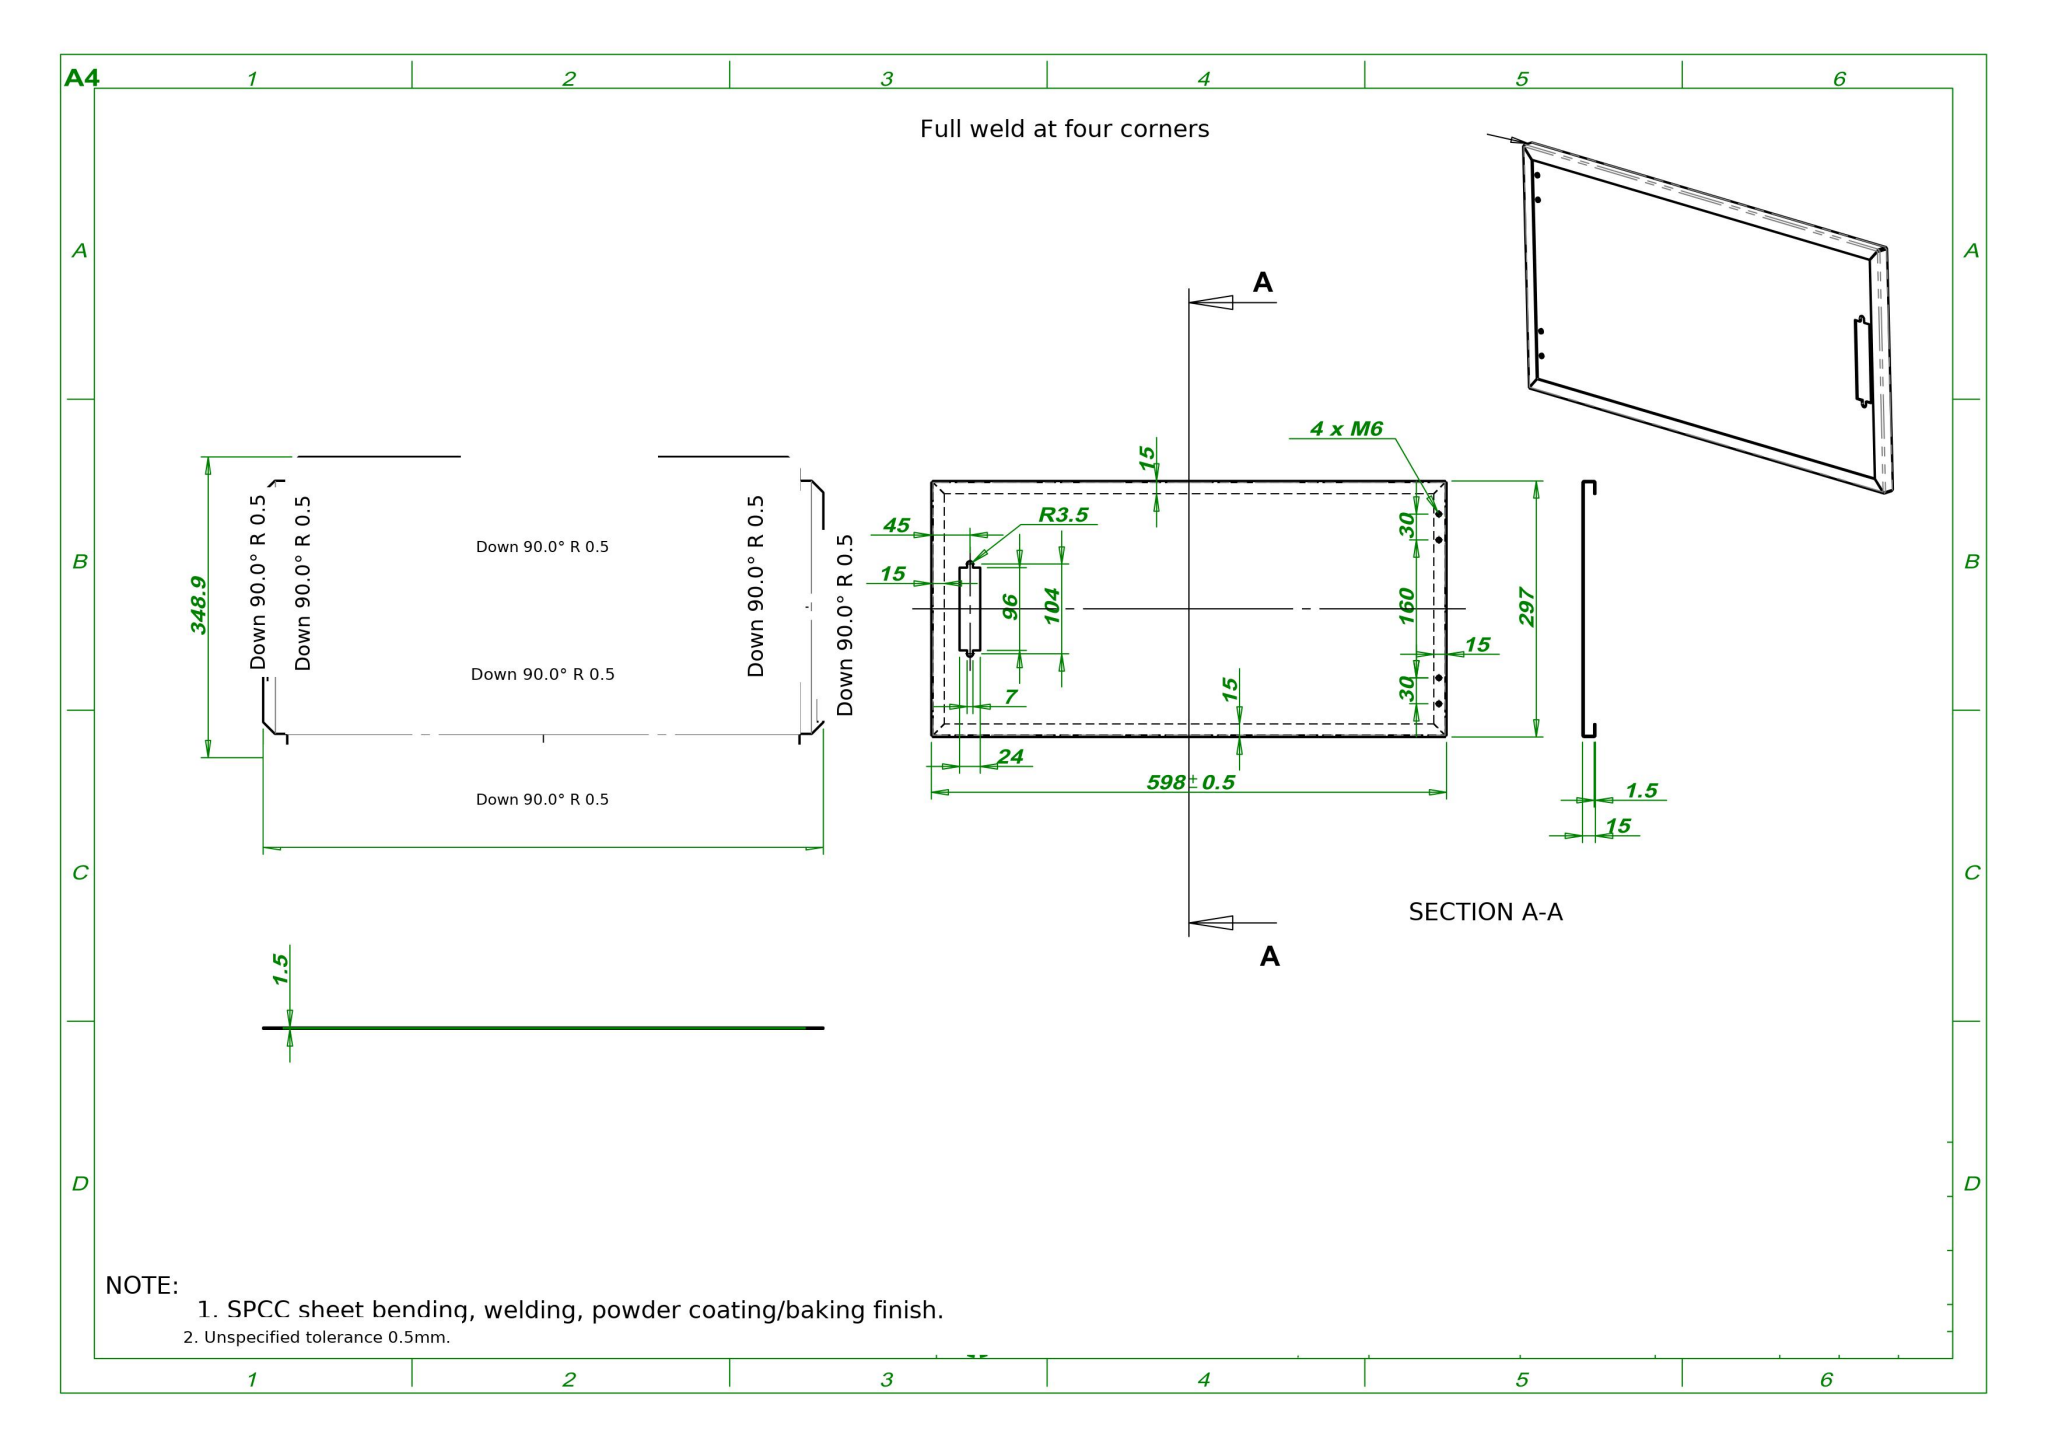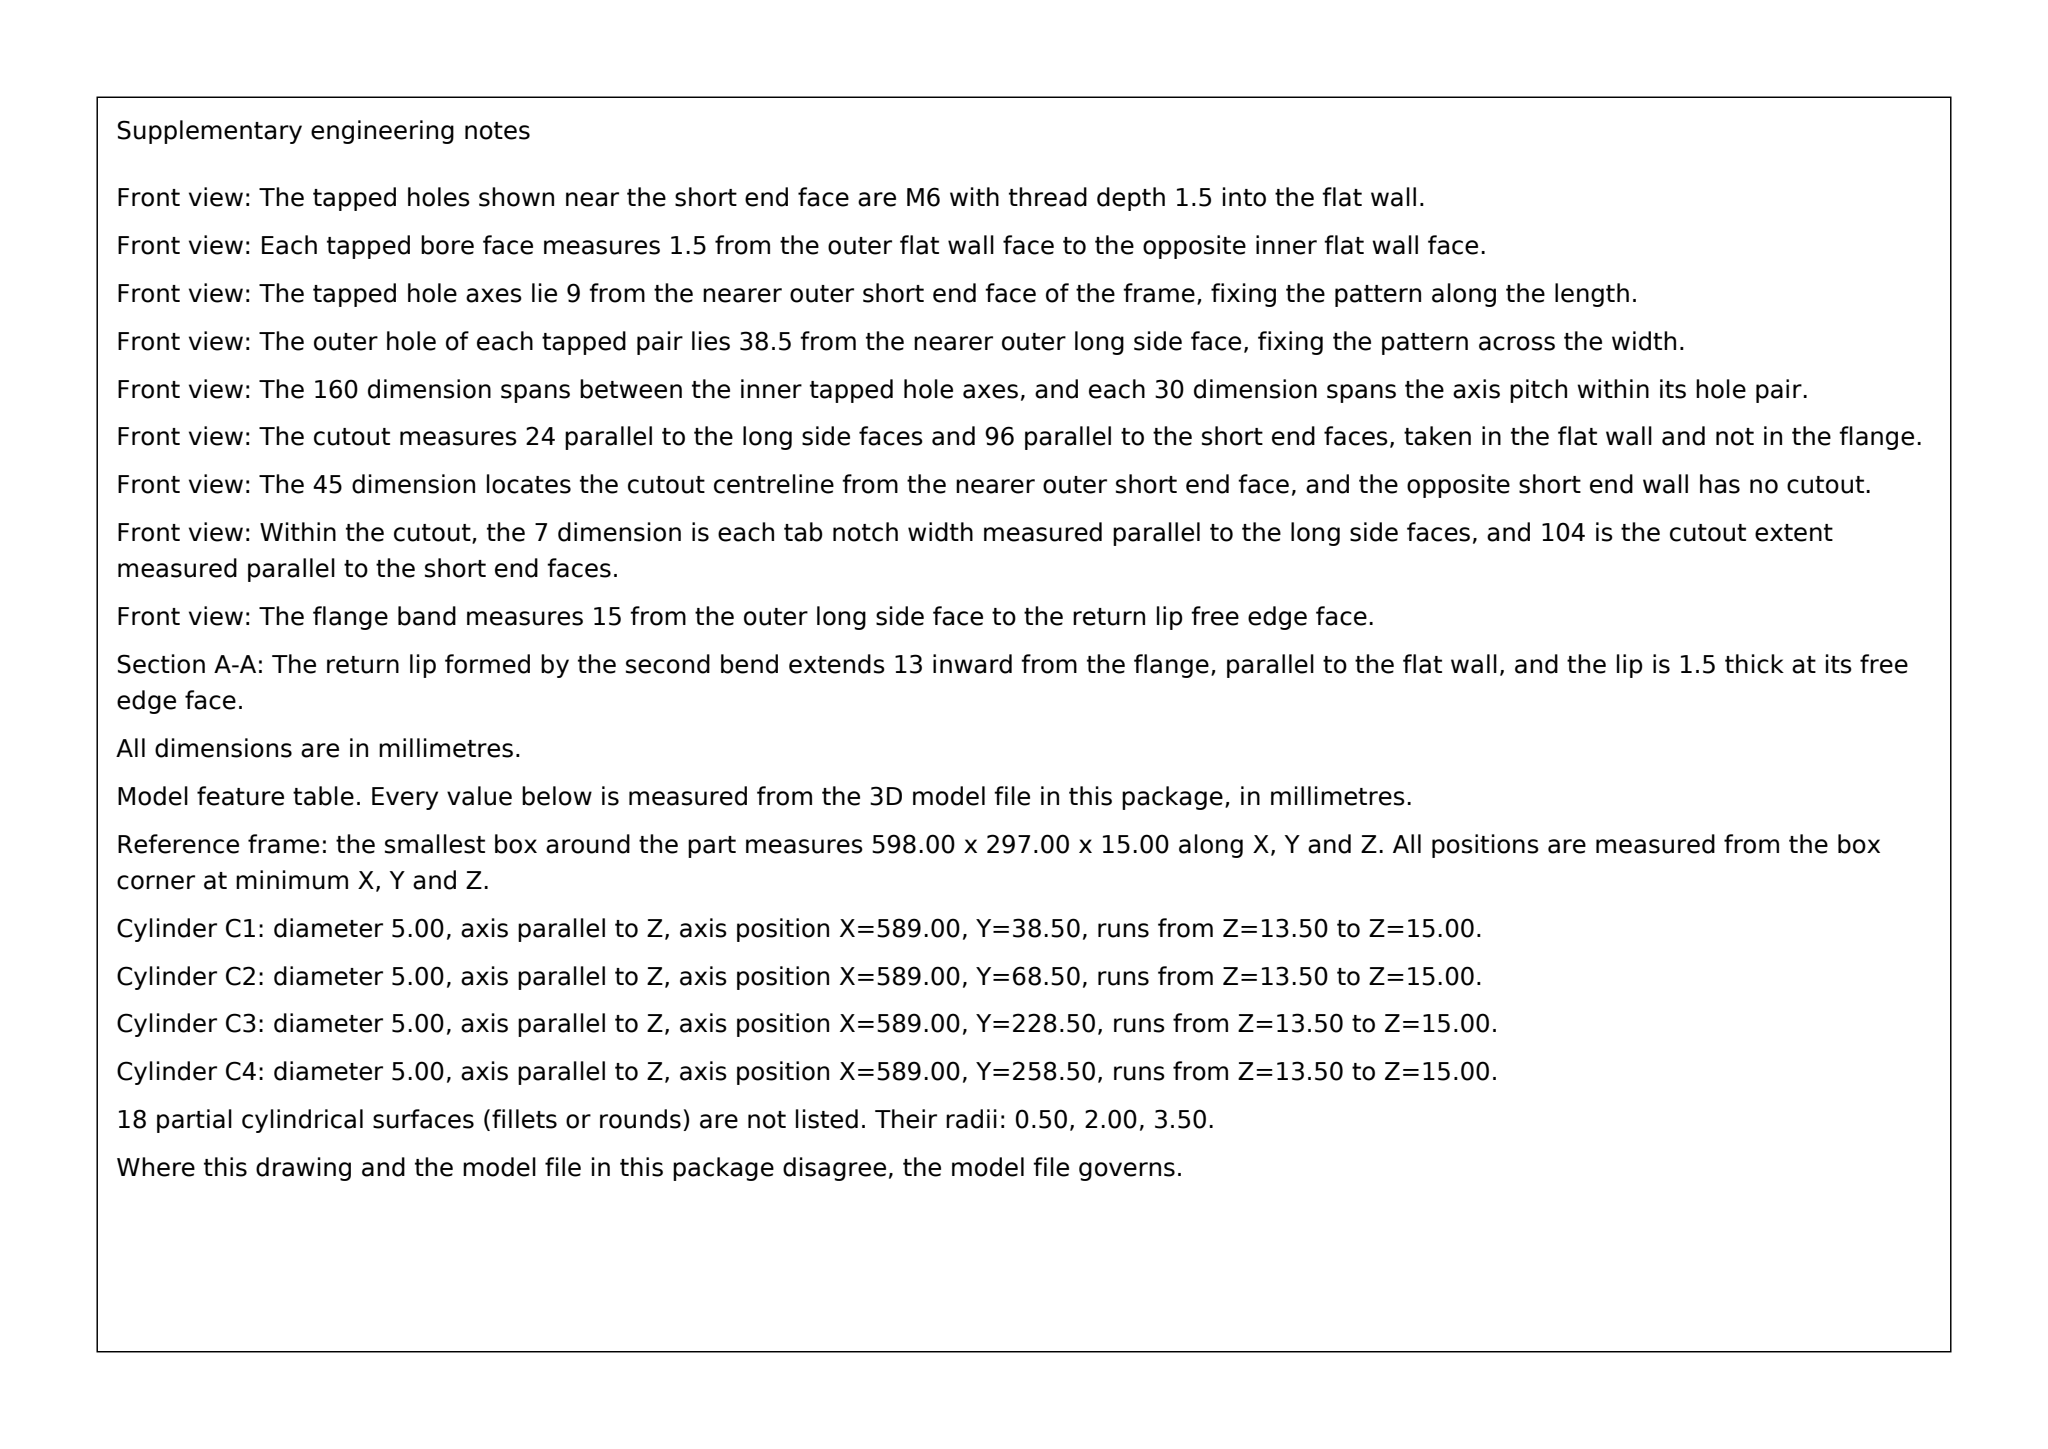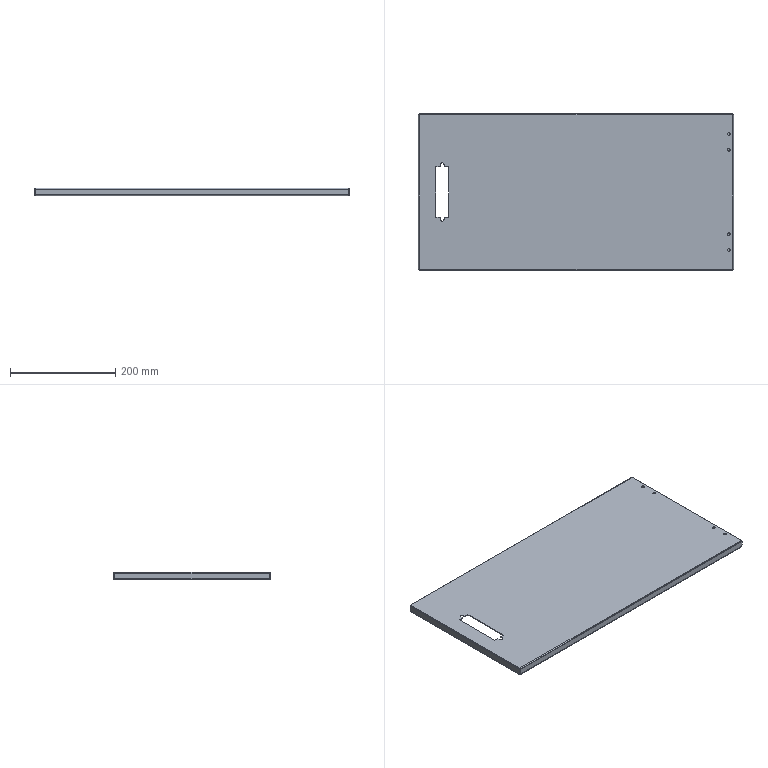Part | SolidWorks | mm | material SPCC | 1 solid | 98 faces | box 598 x 297 x 15 mm | volume 330615 mm3 | plane 56 | cylinder 26 | spline 16 | commonest cylinder face diameters 5 x8 4 x8 1 x8 7 x2
Drawing notes:
FLAT PATTERN OVERALL LENGTH 649.9 (DEVELOPED) | from the solid: Outer box 598 long; 4 bend legs 15 ea (x walls 0-1.5/596.5-598, returns to x=15/583); 598+4x15-4x2.025 BD = 649.9, matching 297+51.9=348.9 width
4 x M6: CL 9 FROM RH EDGE, 30 & 160 SPACING (SEE VIEW) | from the solid: Ø5 z-holes at x=589 (598-589=9 from right edge), y=38.5/68.5/228.5/258.5 -> 30 and 160 pitches